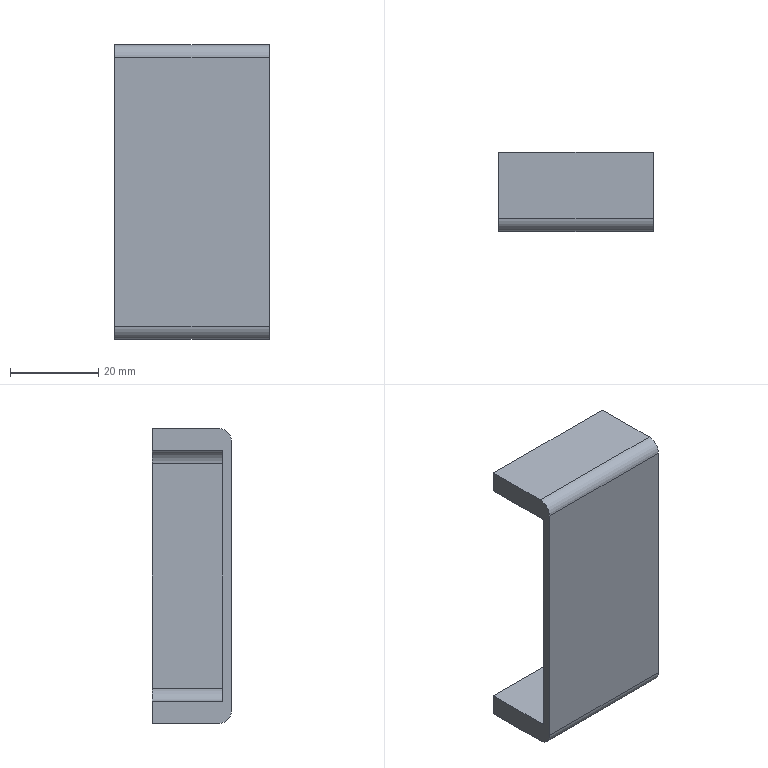CAM job | Mastercam | mm | 16 operations | part box 35 x 18 x 67
1. Facing | 1 - 50 J面铣
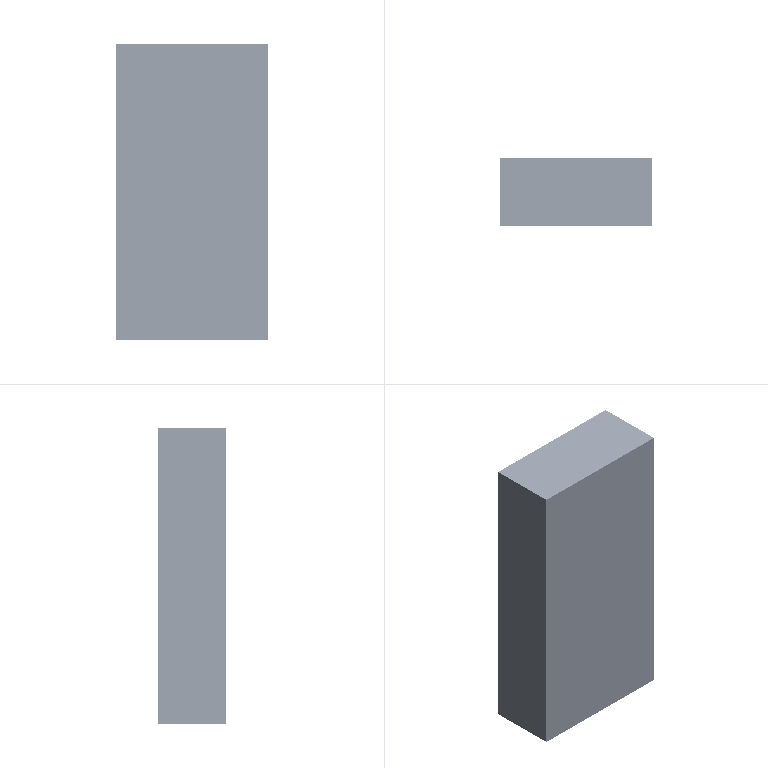2. 2D High Speed (2D Dynamic Mill) | 9 - 10C 平底刀
3. 2D High Speed (2D Dynamic Mill) | 9 - 10C 平底刀
4. Contour (Remachining) | 6 - 6 平底刀
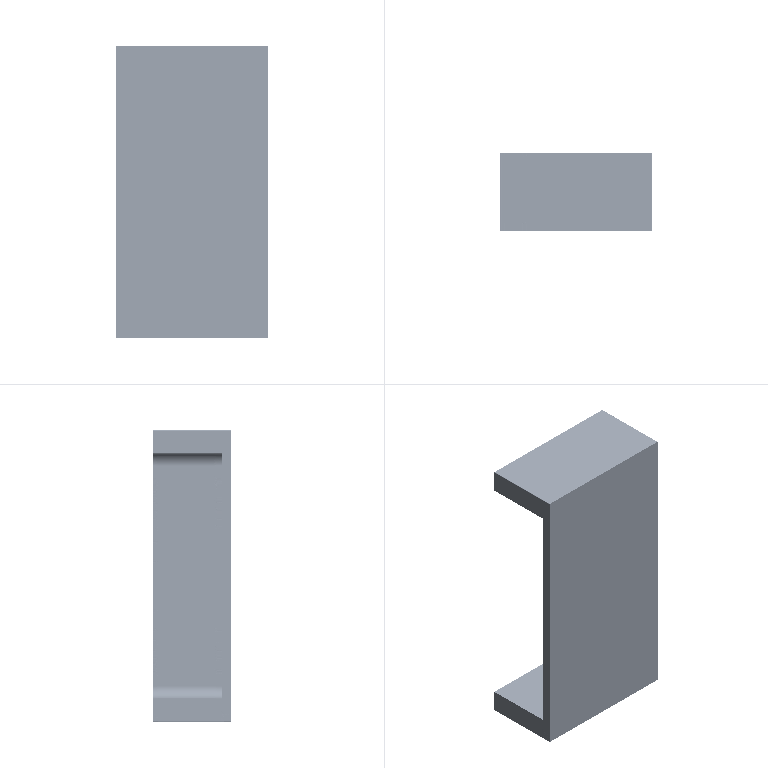5. Drill/Counterbore | 2 - 6定位倒角
6. Peck Drill | 12 - 2.5 钻头
7. Thread Mill | 22 - M3/0.5  -D2.4L9螺纹铣刀
8. Facing | 1 - 50 J面铣
9. Contour (2D) | 10 - 10J 平底刀
10. 2D High Speed (2D Area Mill) | 6 - 6 平底刀
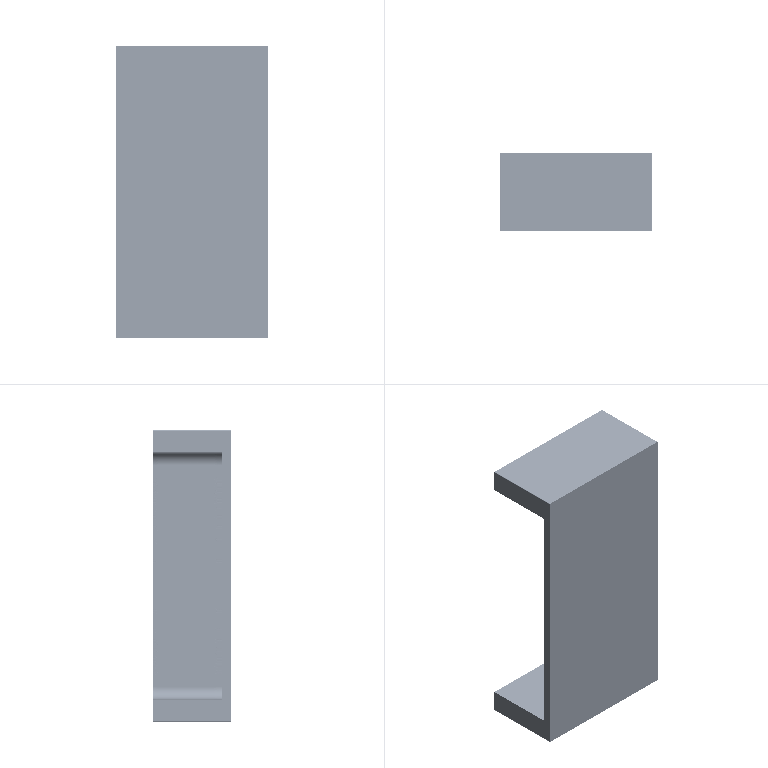11. Contour (2D) | 6 - 6 平底刀
12. Model Chamfer | 2 - 6定位倒角
13. Facing | 9 - 10C 平底刀
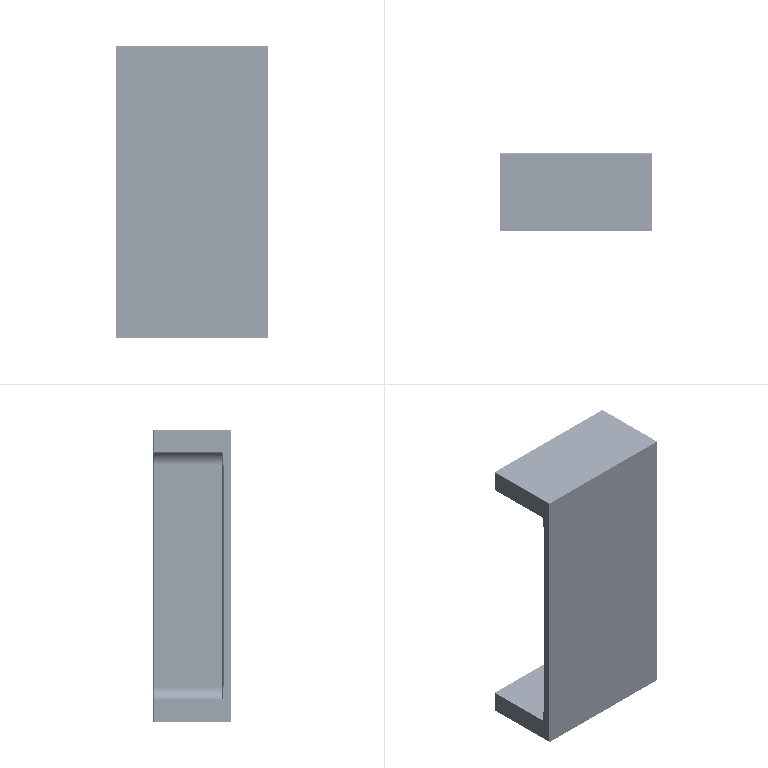14. Facing | 10 - 10J 平底刀
15. Surface Finish Flowline | 3 - 10 -R1.0圆鼻铣刀
16. Contour (2D chamfer) | 2 - 6定位倒角